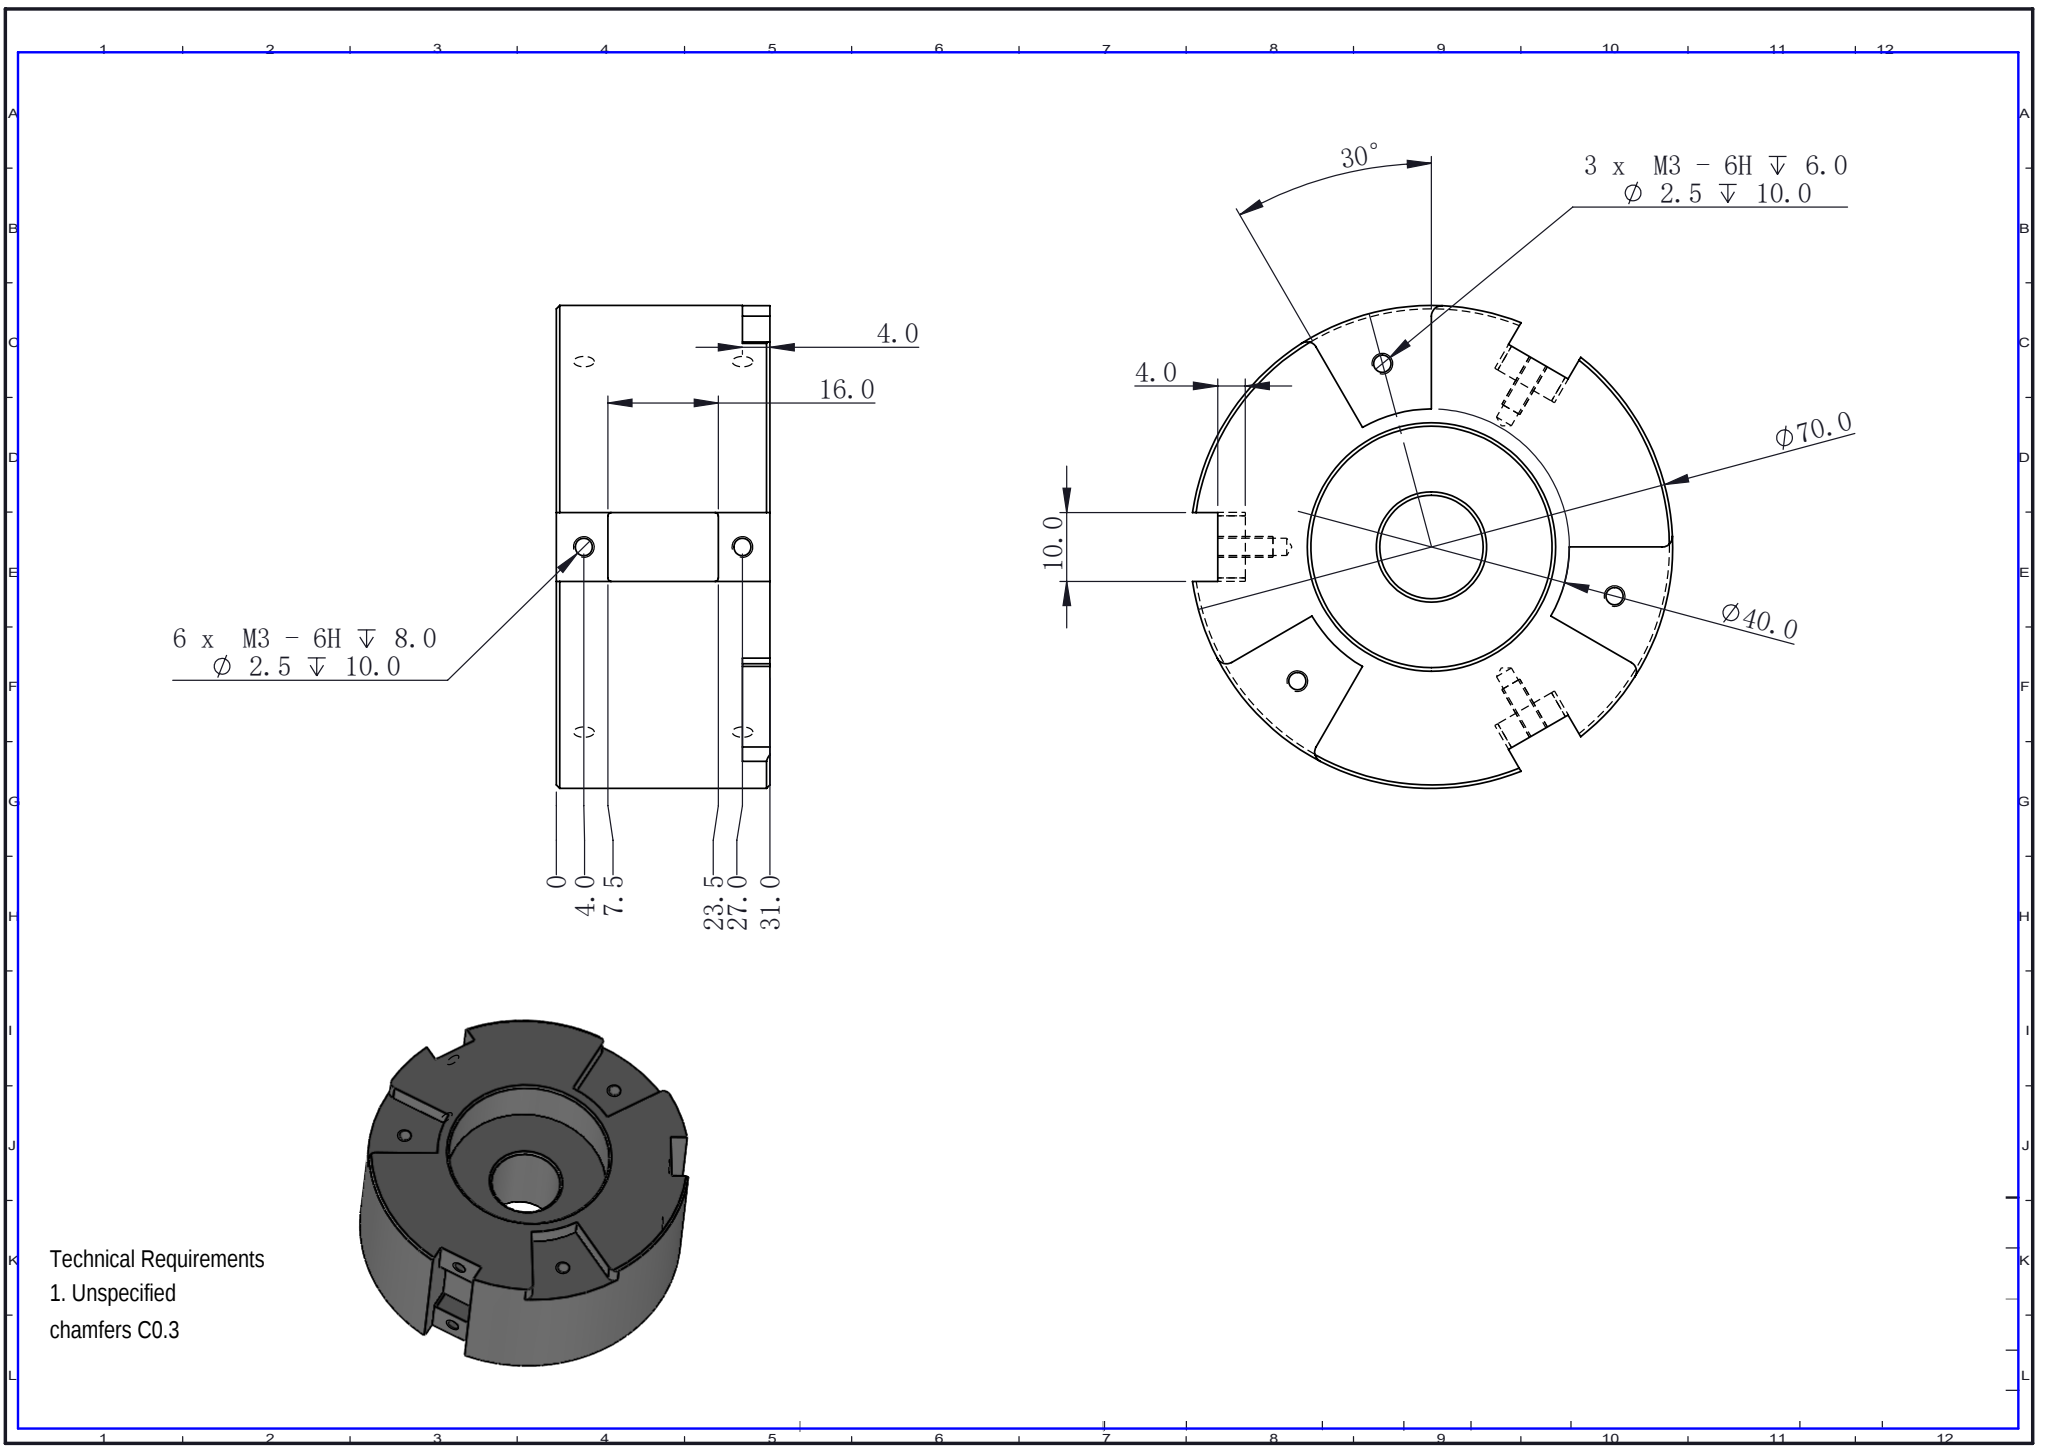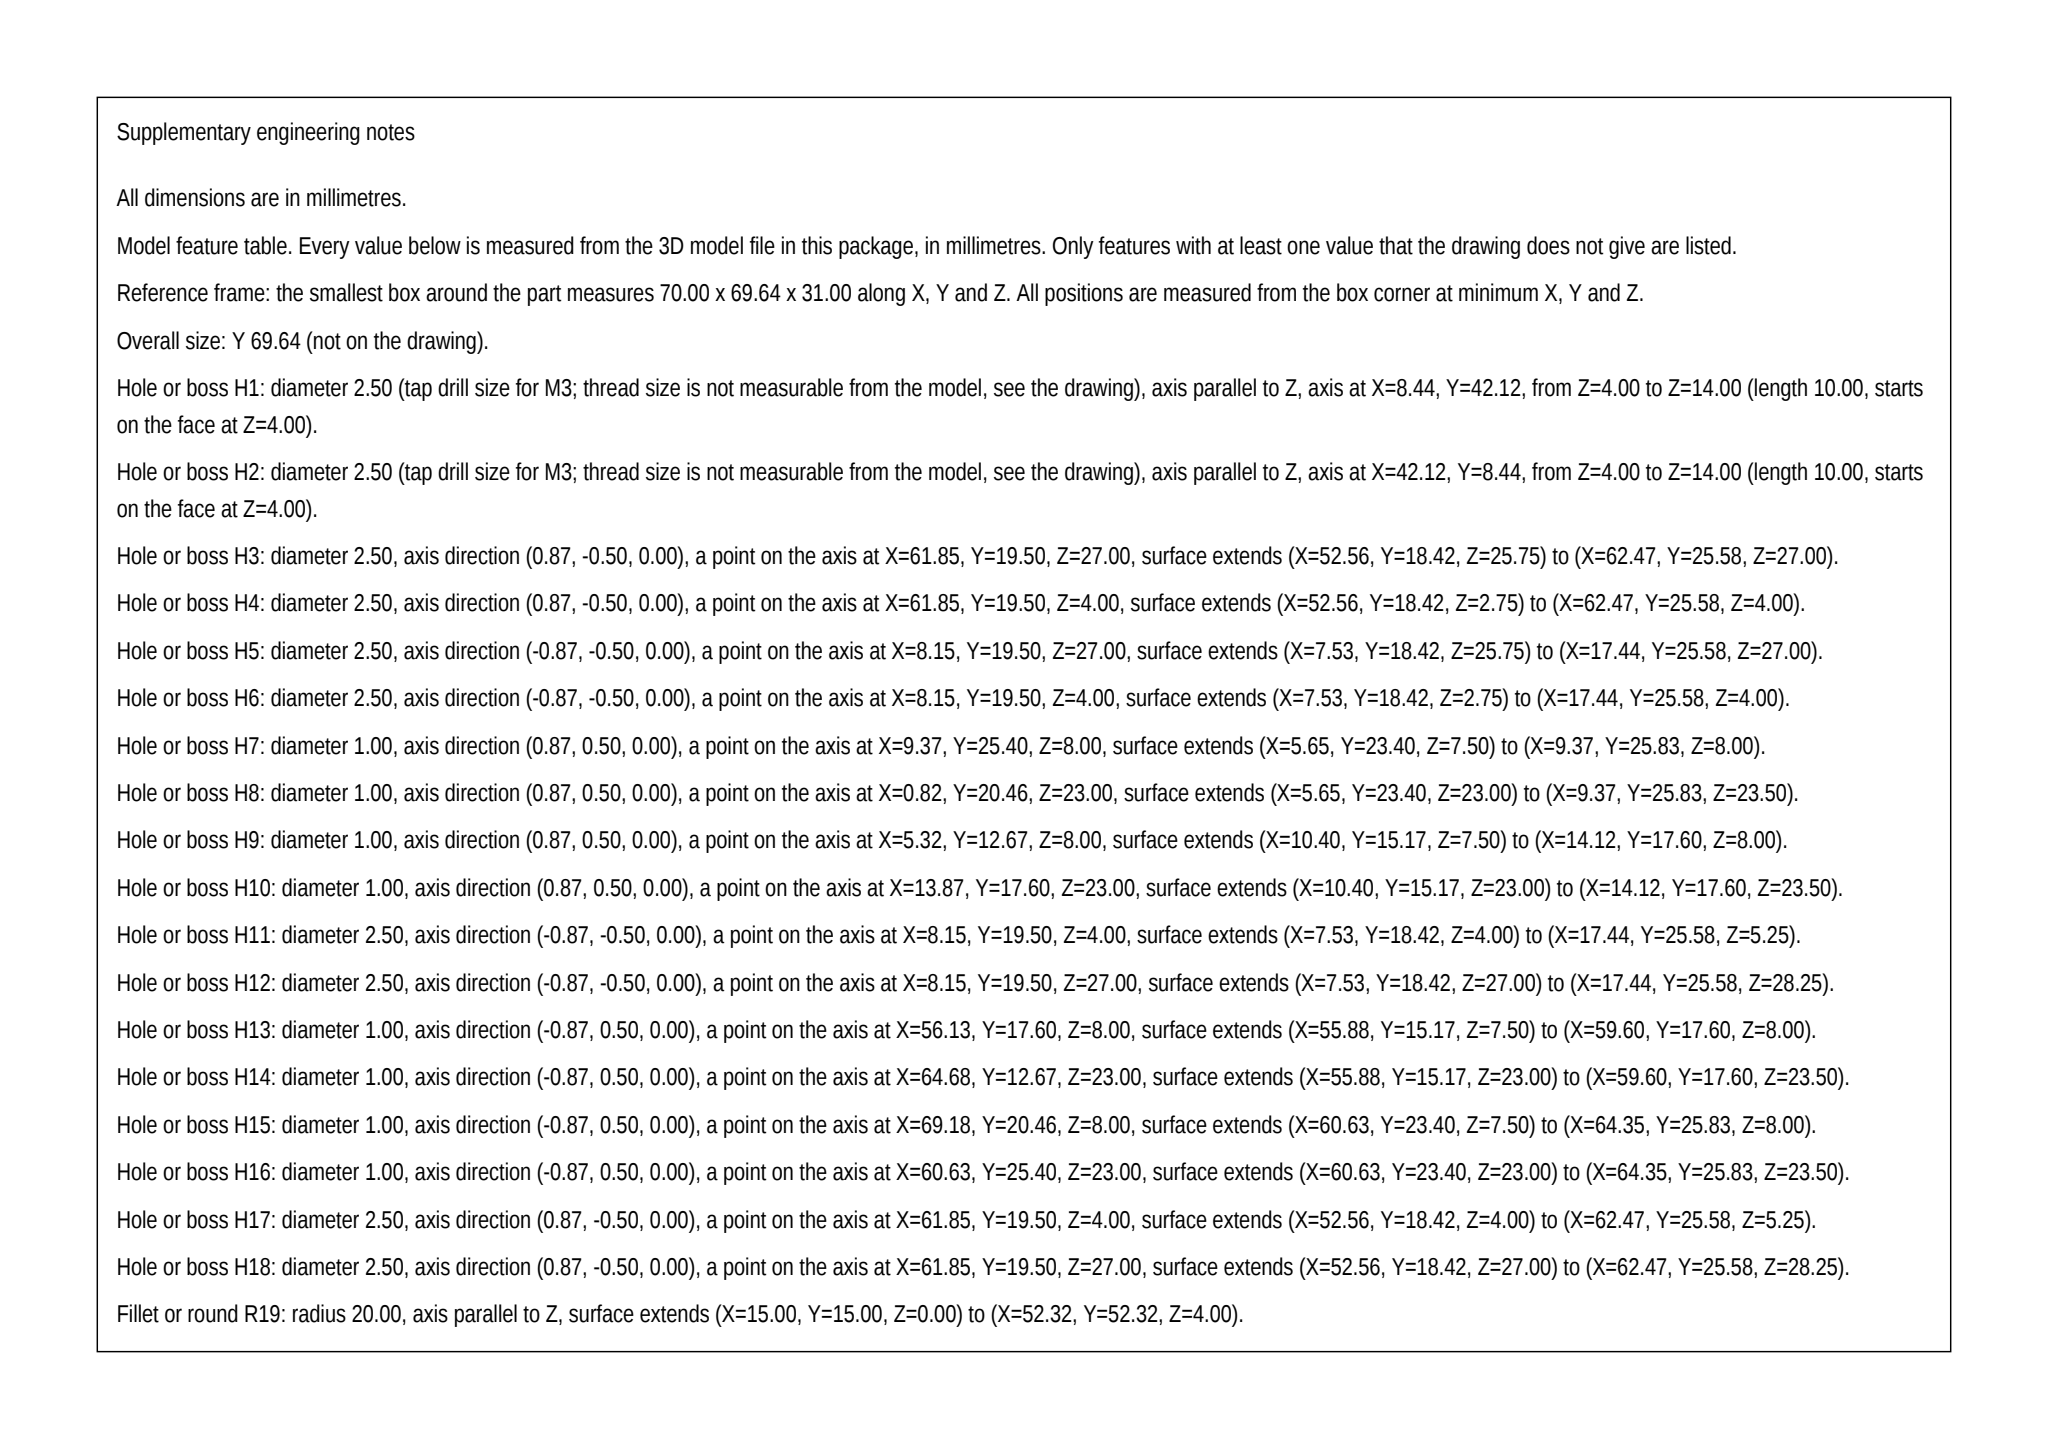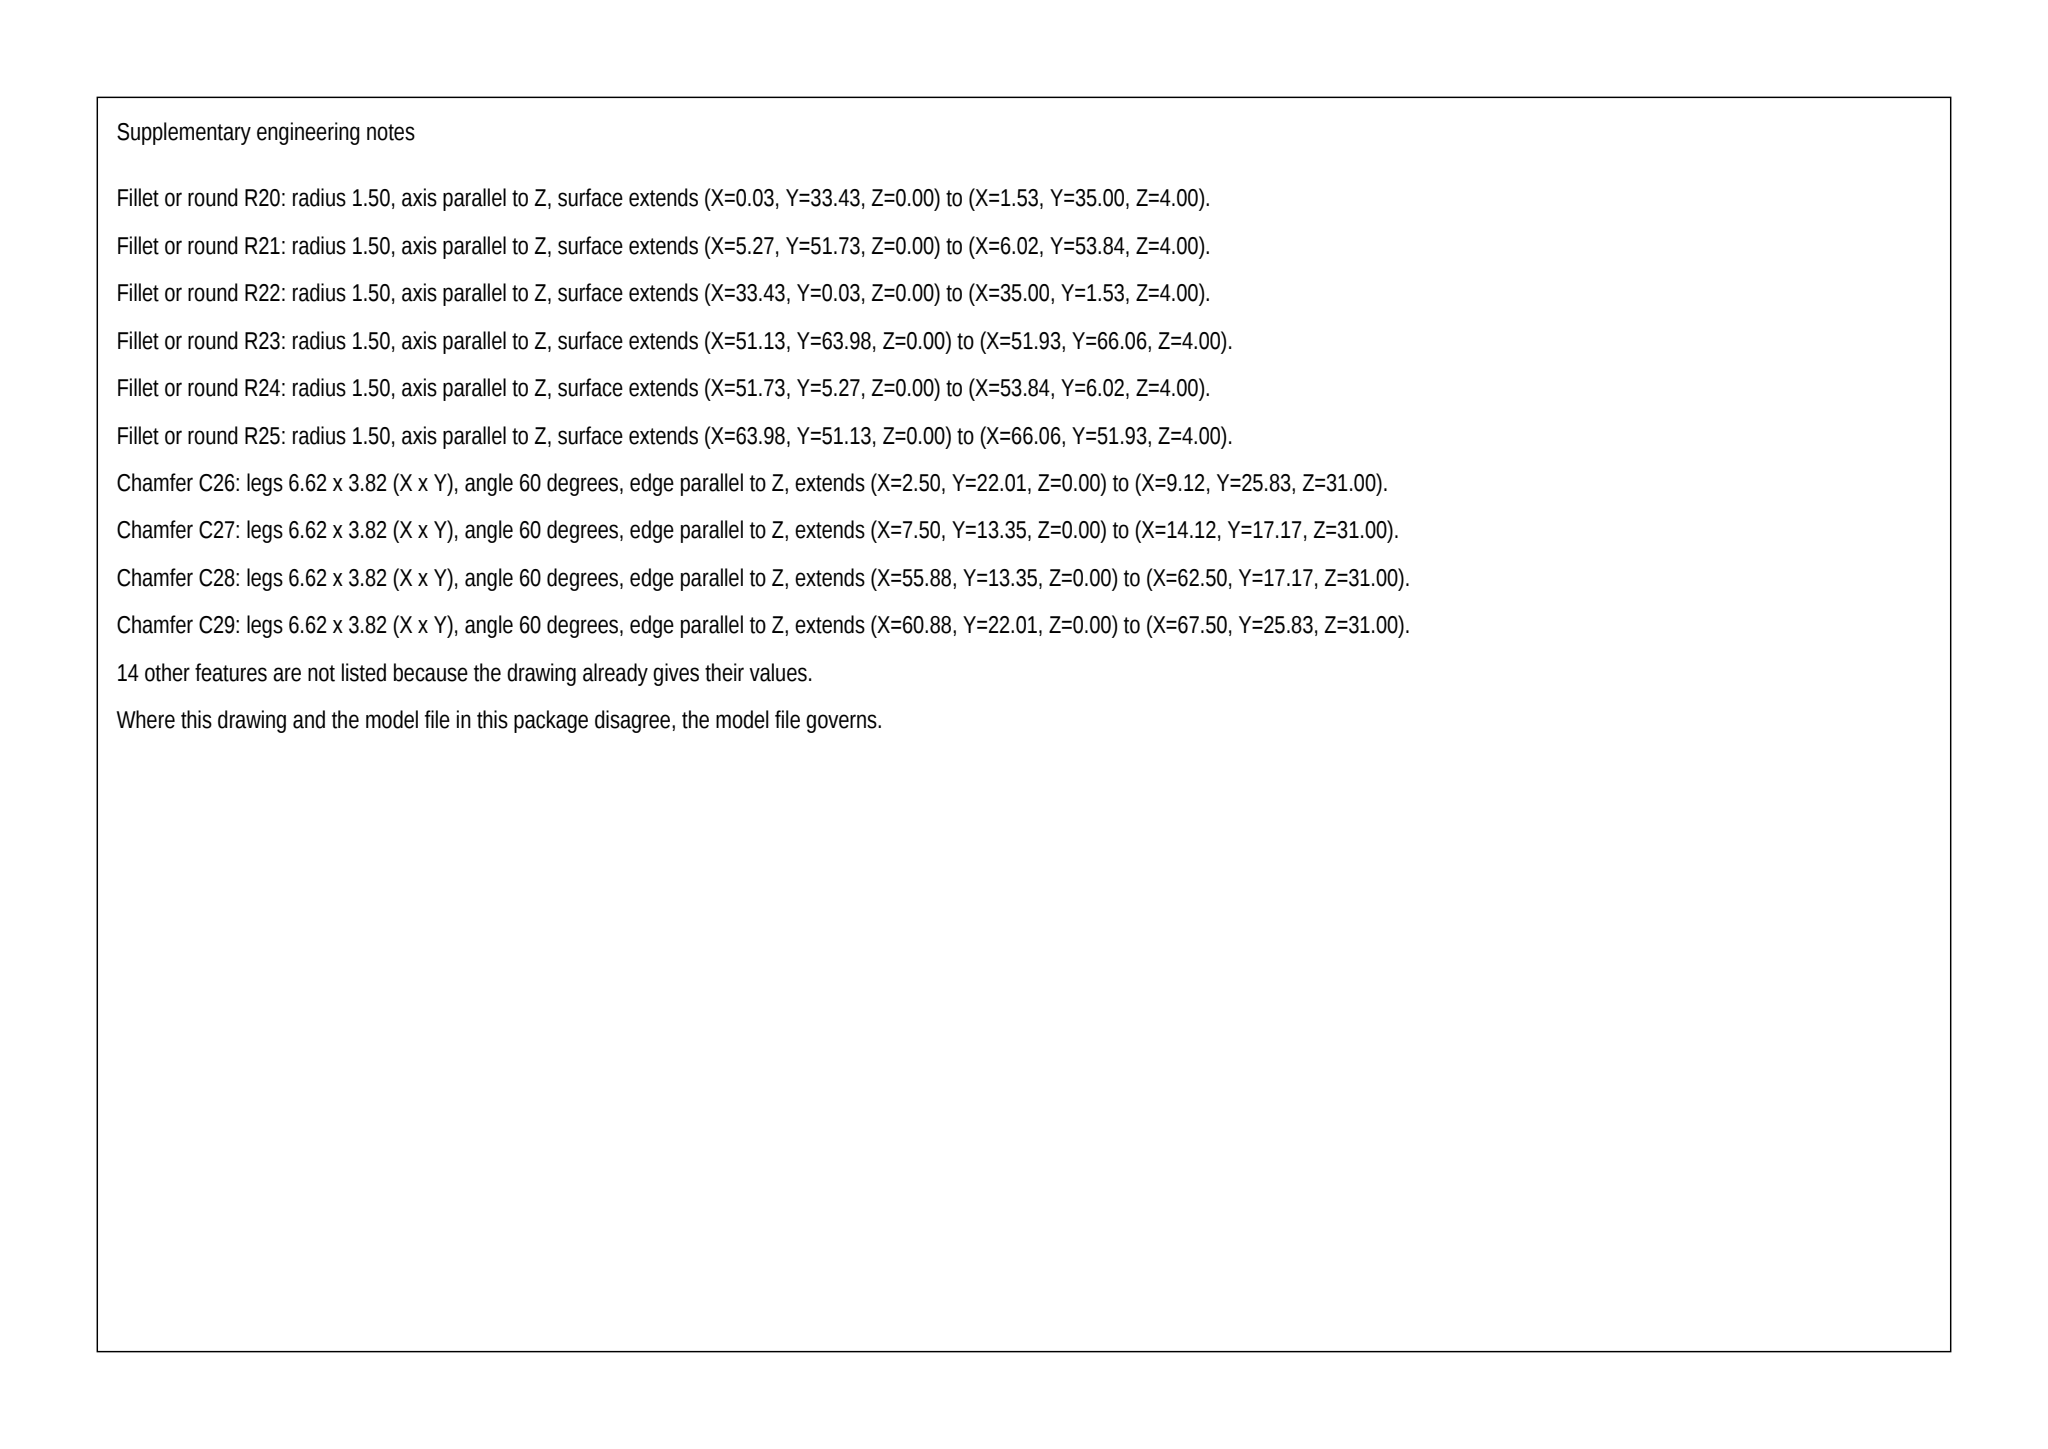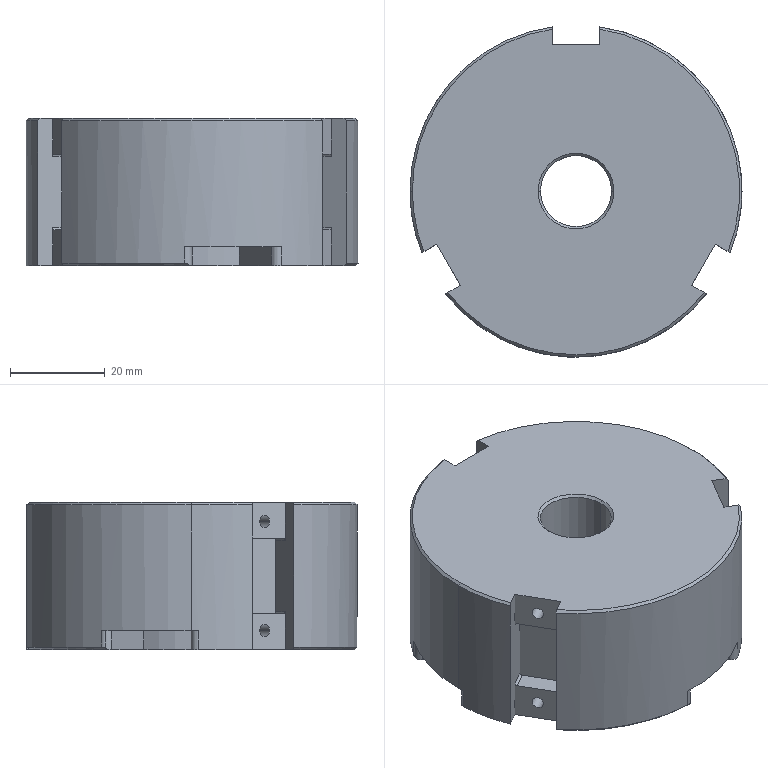Part | SolidWorks | mm | 1 solid | 114 faces | box 70 x 69.64 x 31 mm | volume 96540 mm3 | cylinder 49 | plane 33 | cone 32 | commonest cylinder face diameters 2.5 x18 1 x12 3 x8 70 x4 40 x3 35 x2 15 x2